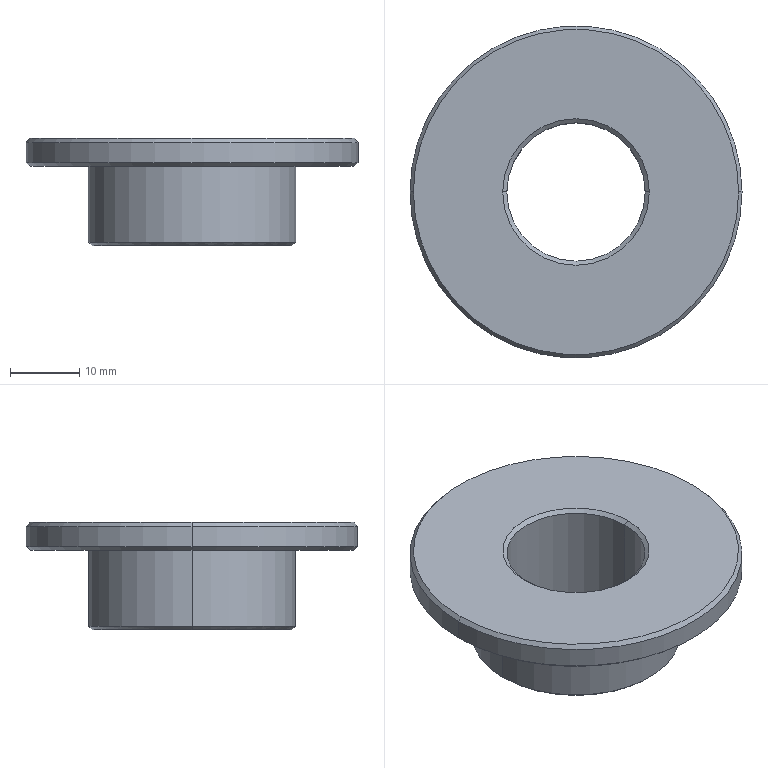Component | SolidWorks | CuttingMotorFixedShaftSleeve-1 | 1 solid | 19 faces | box 48 x 48 x 15.5 mm | volume 10420 mm3 | cone 10 | cylinder 6 | plane 3 | commonest cylinder face diameters 20 x2 30 x2 48 x2
build123d program:
from build123d import *
from OCP.BRepFilletAPI import BRepFilletAPI_MakeChamfer

# Parameters (mm, degrees)
CHAMFER1_SIZE  = 0.5
CHAMFER1_SIZE2 = 0.5959


with BuildPart() as part:
    # Sketch1 → Revolve1 (revolve)
    with BuildSketch(Plane.XY):
        Polygon((24, 0), (24, -4), (15, -4), (15, -15.5), (10, -15.5), (10, 0), align=None)
    revolve(axis=Axis((0, -1263.669, 0), (0, 1, 0)))

    # Chamfer1: one chamfer whose edges measure the first distance from different faces: ONE call of the kernel's chamfer builder (chamfer() names one face for all edges)
    chamfer1_edges_1 = [part.edges().sort_by_distance(p)[0] for p in [
        (-10, 0, 0),
    ]]
    chamfer1_side_1 = [part.faces().sort_by_distance(p)[0] for p in [
        (-10, -7.75, 0),
    ]]
    chamfer1_edges_2 = [part.edges().sort_by_distance(p)[0] for p in [
        (-10, -15.5, 0),
    ]]
    chamfer1_side_2 = [part.faces().sort_by_distance(p)[0] for p in [
        (-14.576, -15.5, 0),
    ]]
    chamfer1_edges_3 = [part.edges().sort_by_distance(p)[0] for p in [
        (-15, -15.5, 0),
    ]]
    chamfer1_side_3 = [part.faces().sort_by_distance(p)[0] for p in [
        (-15, -9.75, 0),
    ]]
    chamfer1_edges_4 = [part.edges().sort_by_distance(p)[0] for p in [
        (-24, -4, 0),
    ]]
    chamfer1_side_4 = [part.faces().sort_by_distance(p)[0] for p in [
        (-24, -2, 0),
    ]]
    chamfer1_edges_5 = [part.edges().sort_by_distance(p)[0] for p in [
        (-24, 0, 0),
    ]]
    chamfer1_side_5 = [part.faces().sort_by_distance(p)[0] for p in [
        (-10.679, 0, 0),
    ]]
    chamfer1 = BRepFilletAPI_MakeChamfer(part.part.solid().wrapped)
    for e in chamfer1_edges_1:
        chamfer1.Add(CHAMFER1_SIZE, CHAMFER1_SIZE2, e.wrapped, chamfer1_side_1[0].wrapped)  # the first distance lies on this face
    for e in chamfer1_edges_2:
        chamfer1.Add(CHAMFER1_SIZE, CHAMFER1_SIZE2, e.wrapped, chamfer1_side_2[0].wrapped)  # the first distance lies on this face
    for e in chamfer1_edges_3:
        chamfer1.Add(CHAMFER1_SIZE, CHAMFER1_SIZE2, e.wrapped, chamfer1_side_3[0].wrapped)  # the first distance lies on this face
    for e in chamfer1_edges_4:
        chamfer1.Add(CHAMFER1_SIZE, CHAMFER1_SIZE2, e.wrapped, chamfer1_side_4[0].wrapped)  # the first distance lies on this face
    for e in chamfer1_edges_5:
        chamfer1.Add(CHAMFER1_SIZE, CHAMFER1_SIZE2, e.wrapped, chamfer1_side_5[0].wrapped)  # the first distance lies on this face
    add(Compound.cast(chamfer1.Shape()), mode=Mode.REPLACE)


solid = part.part

# Placed as in the assembly
solid = solid.moved(Location((-22.772, -46.766, 806), (90, 0, 0)))
STEP:
#1=COLOUR_RGB('',0.7922,0.8196,0.9333);
#2=FILL_AREA_STYLE_COLOUR('',#1);
#3=FILL_AREA_STYLE('',(#2));
#4=SURFACE_STYLE_FILL_AREA(#3);
#5=SURFACE_SIDE_STYLE('',(#4));
#6=SURFACE_STYLE_USAGE(.BOTH.,#5);
#7=PRESENTATION_STYLE_ASSIGNMENT((#6));
#8=CARTESIAN_POINT('',(-1.822,-1.841,31.732));
#9=VERTEX_POINT('',#8);
#10=CARTESIAN_POINT('',(0.02866,-1.841,31.732));
#11=VERTEX_POINT('',#10);
#12=CARTESIAN_POINT('',(-0.8965,-1.841,31.732));
#13=DIRECTION('',(0.,-0.,1.));
#14=DIRECTION('',(-1.,-0.,0.));
#15=AXIS2_PLACEMENT_3D('',#12,#13,#14);
#16=CIRCLE('',#15,0.9252);
#17=EDGE_CURVE('',#9,#11,#16,.T.);
#18=ORIENTED_EDGE('',*,*,#17,.F.);
#19=CARTESIAN_POINT('',(-1.841,-1.841,31.709));
#20=VERTEX_POINT('',#19);
#21=CARTESIAN_POINT('',(-1.841,-1.841,31.709));
#22=DIRECTION('',(-0.6428,-0.,-0.766));
#23=VECTOR('',#22,39.37);
#24=LINE('',#21,#23);
#25=EDGE_CURVE('',#9,#20,#24,.T.);
#26=ORIENTED_EDGE('',*,*,#25,.T.);
#27=CARTESIAN_POINT('',(0.04834,-1.841,31.709));
#28=VERTEX_POINT('',#27);
#29=CARTESIAN_POINT('',(-0.8965,-1.841,31.709));
#30=DIRECTION('',(-0.,0.,-1.));
#31=DIRECTION('',(-1.,-0.,0.));
#32=AXIS2_PLACEMENT_3D('',#29,#30,#31);
#33=CIRCLE('',#32,0.9449);
#34=EDGE_CURVE('',#28,#20,#33,.T.);
#35=ORIENTED_EDGE('',*,*,#34,.F.);
#36=CARTESIAN_POINT('',(0.04834,-1.841,31.709));
#37=DIRECTION('',(0.6428,0.,-0.766));
#38=VECTOR('',#37,39.37);
#39=LINE('',#36,#38);
#40=EDGE_CURVE('',#11,#28,#39,.T.);
#41=ORIENTED_EDGE('',*,*,#40,.F.);
#42=EDGE_LOOP('',(#18,#26,#35,#41));
#43=FACE_OUTER_BOUND('',#42,.T.);
#44=CARTESIAN_POINT('',(-0.8965,-1.841,31.709));
#45=DIRECTION('',(-0.,0.,-1.));
#46=DIRECTION('',(1.,0.,0.));
#47=AXIS2_PLACEMENT_3D('',#44,#45,#46);
#48=CONICAL_SURFACE('',#47,0.9449,0.6981);
#49=ADVANCED_FACE('',(#43),#48,.T.);
#50=CARTESIAN_POINT('',(0.02488,-1.841,31.575));
#51=VERTEX_POINT('',#50);
#52=CARTESIAN_POINT('',(-1.818,-1.841,31.575));
#53=VERTEX_POINT('',#52);
#54=CARTESIAN_POINT('',(-0.8965,-1.841,31.575));
#55=DIRECTION('',(-0.,0.,-1.));
#56=DIRECTION('',(1.,0.,0.));
#57=AXIS2_PLACEMENT_3D('',#54,#55,#56);
#58=CIRCLE('',#57,0.9214);
#59=EDGE_CURVE('',#51,#53,#58,.T.);
#60=ORIENTED_EDGE('',*,*,#59,.F.);
#61=CARTESIAN_POINT('',(0.04834,-1.841,31.594));
#62=VERTEX_POINT('',#61);
#63=CARTESIAN_POINT('',(0.02488,-1.841,31.575));
#64=DIRECTION('',(0.766,0.,0.6428));
#65=VECTOR('',#64,39.37);
#66=LINE('',#63,#65);
#67=EDGE_CURVE('',#51,#62,#66,.T.);
#68=ORIENTED_EDGE('',*,*,#67,.T.);
#69=CARTESIAN_POINT('',(-1.841,-1.841,31.594));
#70=VERTEX_POINT('',#69);
#71=CARTESIAN_POINT('',(-0.8965,-1.841,31.594));
#72=DIRECTION('',(0.,-0.,1.));
#73=DIRECTION('',(1.,0.,0.));
#74=AXIS2_PLACEMENT_3D('',#71,#72,#73);
#75=CIRCLE('',#74,0.9449);
#76=EDGE_CURVE('',#70,#62,#75,.T.);
#77=ORIENTED_EDGE('',*,*,#76,.F.);
#78=CARTESIAN_POINT('',(-1.818,-1.841,31.575));
#79=DIRECTION('',(-0.766,-0.,0.6428));
#80=VECTOR('',#79,39.37);
#81=LINE('',#78,#80);
#82=EDGE_CURVE('',#53,#70,#81,.T.);
#83=ORIENTED_EDGE('',*,*,#82,.F.);
#84=EDGE_LOOP('',(#60,#68,#77,#83));
#85=FACE_OUTER_BOUND('',#84,.T.);
#86=CARTESIAN_POINT('',(-0.8965,-1.841,31.575));
#87=DIRECTION('',(0.,-0.,1.));
#88=DIRECTION('',(-1.,-0.,0.));
#89=AXIS2_PLACEMENT_3D('',#86,#87,#88);
#90=CONICAL_SURFACE('',#89,0.9214,0.8727);
#91=ADVANCED_FACE('',(#85),#90,.T.);
#92=CARTESIAN_POINT('',(-0.3294,-1.841,31.122));
#93=VERTEX_POINT('',#92);
#94=CARTESIAN_POINT('',(-1.464,-1.841,31.122));
#95=VERTEX_POINT('',#94);
#96=CARTESIAN_POINT('',(-0.8965,-1.841,31.122));
#97=DIRECTION('',(-0.,0.,-1.));
#98=DIRECTION('',(1.,0.,0.));
#99=AXIS2_PLACEMENT_3D('',#96,#97,#98);
#100=CIRCLE('',#99,0.5671);
#101=EDGE_CURVE('',#93,#95,#100,.T.);
#102=ORIENTED_EDGE('',*,*,#101,.F.);
#103=CARTESIAN_POINT('',(-0.306,-1.841,31.142));
#104=VERTEX_POINT('',#103);
#105=CARTESIAN_POINT('',(-0.3294,-1.841,31.122));
#106=DIRECTION('',(0.766,0.,0.6428));
#107=VECTOR('',#106,39.37);
#108=LINE('',#105,#107);
#109=EDGE_CURVE('',#93,#104,#108,.T.);
#110=ORIENTED_EDGE('',*,*,#109,.T.);
#111=CARTESIAN_POINT('',(-1.487,-1.841,31.142));
#112=VERTEX_POINT('',#111);
#113=CARTESIAN_POINT('',(-0.8965,-1.841,31.142));
#114=DIRECTION('',(0.,-0.,1.));
#115=DIRECTION('',(1.,0.,0.));
#116=AXIS2_PLACEMENT_3D('',#113,#114,#115);
#117=CIRCLE('',#116,0.5906);
#118=EDGE_CURVE('',#112,#104,#117,.T.);
#119=ORIENTED_EDGE('',*,*,#118,.F.);
#120=CARTESIAN_POINT('',(-1.464,-1.841,31.122));
#121=DIRECTION('',(-0.766,-0.,0.6428));
#122=VECTOR('',#121,39.37);
#123=LINE('',#120,#122);
#124=EDGE_CURVE('',#95,#112,#123,.T.);
#125=ORIENTED_EDGE('',*,*,#124,.F.);
#126=EDGE_LOOP('',(#102,#110,#119,#125));
#127=FACE_OUTER_BOUND('',#126,.T.);
#128=CARTESIAN_POINT('',(-0.8965,-1.841,31.122));
#129=DIRECTION('',(0.,-0.,1.));
#130=DIRECTION('',(-1.,-0.,0.));
#131=AXIS2_PLACEMENT_3D('',#128,#129,#130);
#132=CONICAL_SURFACE('',#131,0.5671,0.8727);
#133=ADVANCED_FACE('',(#127),#132,.T.);
#134=CARTESIAN_POINT('',(-1.29,-1.841,31.146));
#135=VERTEX_POINT('',#134);
#136=CARTESIAN_POINT('',(-0.5028,-1.841,31.146));
#137=VERTEX_POINT('',#136);
#138=CARTESIAN_POINT('',(-0.8965,-1.841,31.146));
#139=DIRECTION('',(-0.,0.,-1.));
#140=DIRECTION('',(1.,0.,0.));
#141=AXIS2_PLACEMENT_3D('',#138,#139,#140);
#142=CIRCLE('',#141,0.3937);
#143=EDGE_CURVE('',#135,#137,#142,.T.);
#144=ORIENTED_EDGE('',*,*,#143,.F.);
#145=CARTESIAN_POINT('',(-1.31,-1.841,31.122));
#146=VERTEX_POINT('',#145);
#147=CARTESIAN_POINT('',(-1.29,-1.841,31.146));
#148=DIRECTION('',(-0.6428,-0.,-0.766));
#149=VECTOR('',#148,39.37);
#150=LINE('',#147,#149);
#151=EDGE_CURVE('',#135,#146,#150,.T.);
#152=ORIENTED_EDGE('',*,*,#151,.T.);
#153=CARTESIAN_POINT('',(-0.4832,-1.841,31.122));
#154=VERTEX_POINT('',#153);
#155=CARTESIAN_POINT('',(-0.8965,-1.841,31.122));
#156=DIRECTION('',(0.,-0.,1.));
#157=DIRECTION('',(1.,0.,0.));
#158=AXIS2_PLACEMENT_3D('',#155,#156,#157);
#159=CIRCLE('',#158,0.4134);
#160=EDGE_CURVE('',#154,#146,#159,.T.);
#161=ORIENTED_EDGE('',*,*,#160,.F.);
#162=CARTESIAN_POINT('',(-0.5028,-1.841,31.146));
#163=DIRECTION('',(0.6428,0.,-0.766));
#164=VECTOR('',#163,39.37);
#165=LINE('',#162,#164);
#166=EDGE_CURVE('',#137,#154,#165,.T.);
#167=ORIENTED_EDGE('',*,*,#166,.F.);
#168=EDGE_LOOP('',(#144,#152,#161,#167));
#169=FACE_OUTER_BOUND('',#168,.T.);
#170=CARTESIAN_POINT('',(-0.8965,-1.841,31.146));
#171=DIRECTION('',(-0.,0.,-1.));
#172=DIRECTION('',(1.,0.,0.));
#173=AXIS2_PLACEMENT_3D('',#170,#171,#172);
#174=CONICAL_SURFACE('',#173,0.3937,0.6981);
#175=ADVANCED_FACE('',(#169),#174,.F.);
#176=CARTESIAN_POINT('',(-0.5028,-1.841,31.713));
#177=VERTEX_POINT('',#176);
#178=CARTESIAN_POINT('',(-1.29,-1.841,31.713));
#179=VERTEX_POINT('',#178);
#180=CARTESIAN_POINT('',(-0.8965,-1.841,31.713));
#181=DIRECTION('',(0.,-0.,1.));
#182=DIRECTION('',(-1.,-0.,0.));
#183=AXIS2_PLACEMENT_3D('',#180,#181,#182);
#184=CIRCLE('',#183,0.3937);
#185=EDGE_CURVE('',#177,#179,#184,.T.);
#186=ORIENTED_EDGE('',*,*,#185,.F.);
#187=CARTESIAN_POINT('',(-0.4794,-1.841,31.732));
#188=VERTEX_POINT('',#187);
#189=CARTESIAN_POINT('',(-0.4794,-1.841,31.732));
#190=DIRECTION('',(0.766,0.,0.6428));
#191=VECTOR('',#190,39.37);
#192=LINE('',#189,#191);
#193=EDGE_CURVE('',#177,#188,#192,.T.);
#194=ORIENTED_EDGE('',*,*,#193,.T.);
#195=CARTESIAN_POINT('',(-1.314,-1.841,31.732));
#196=VERTEX_POINT('',#195);
#197=CARTESIAN_POINT('',(-0.8965,-1.841,31.732));
#198=DIRECTION('',(-0.,0.,-1.));
#199=DIRECTION('',(-1.,-0.,0.));
#200=AXIS2_PLACEMENT_3D('',#197,#198,#199);
#201=CIRCLE('',#200,0.4172);
#202=EDGE_CURVE('',#196,#188,#201,.T.);
#203=ORIENTED_EDGE('',*,*,#202,.F.);
#204=CARTESIAN_POINT('',(-1.314,-1.841,31.732));
#205=DIRECTION('',(-0.766,-0.,0.6428));
#206=VECTOR('',#205,39.37);
#207=LINE('',#204,#206);
#208=EDGE_CURVE('',#179,#196,#207,.T.);
#209=ORIENTED_EDGE('',*,*,#208,.F.);
#210=EDGE_LOOP('',(#186,#194,#203,#209));
#211=FACE_OUTER_BOUND('',#210,.T.);
#212=CARTESIAN_POINT('',(-0.8965,-1.841,31.732));
#213=DIRECTION('',(0.,-0.,1.));
#214=DIRECTION('',(-1.,-0.,0.));
#215=AXIS2_PLACEMENT_3D('',#212,#213,#214);
#216=CONICAL_SURFACE('',#215,0.4172,0.8727);
#217=ADVANCED_FACE('',(#211),#216,.F.);
#218=ORIENTED_EDGE('',*,*,#185,.T.);
#219=CARTESIAN_POINT('',(-1.29,-1.841,-18.018));
#220=DIRECTION('',(-0.,0.,-1.));
#221=VECTOR('',#220,39.37);
#222=LINE('',#219,#221);
#223=EDGE_CURVE('',#179,#135,#222,.T.);
#224=ORIENTED_EDGE('',*,*,#223,.T.);
#225=ORIENTED_EDGE('',*,*,#143,.T.);
#226=CARTESIAN_POINT('',(-0.5028,-1.841,-18.018));
#227=DIRECTION('',(-0.,0.,-1.));
#228=VECTOR('',#227,39.37);
#229=LINE('',#226,#228);
#230=EDGE_CURVE('',#177,#137,#229,.T.);
#231=ORIENTED_EDGE('',*,*,#230,.F.);
#232=EDGE_LOOP('',(#218,#224,#225,#231));
#233=FACE_OUTER_BOUND('',#232,.T.);
#234=CARTESIAN_POINT('',(-0.8965,-1.841,-18.018));
#235=DIRECTION('',(-0.,0.,-1.));
#236=DIRECTION('',(1.,0.,0.));
#237=AXIS2_PLACEMENT_3D('',#234,#235,#236);
#238=CYLINDRICAL_SURFACE('',#237,0.3937);
#239=ADVANCED_FACE('',(#233),#238,.F.);
#240=CARTESIAN_POINT('',(-0.306,-1.841,31.575));
#241=VERTEX_POINT('',#240);
#242=CARTESIAN_POINT('',(-1.487,-1.841,31.575));
#243=VERTEX_POINT('',#242);
#244=CARTESIAN_POINT('',(-0.8965,-1.841,31.575));
#245=DIRECTION('',(-0.,0.,-1.));
#246=DIRECTION('',(1.,0.,0.));
#247=AXIS2_PLACEMENT_3D('',#244,#245,#246);
#248=CIRCLE('',#247,0.5906);
#249=EDGE_CURVE('',#241,#243,#248,.T.);
#250=ORIENTED_EDGE('',*,*,#249,.T.);
#251=CARTESIAN_POINT('',(-1.487,-1.841,-18.018));
#252=DIRECTION('',(-0.,0.,-1.));
#253=VECTOR('',#252,39.37);
#254=LINE('',#251,#253);
#255=EDGE_CURVE('',#243,#112,#254,.T.);
#256=ORIENTED_EDGE('',*,*,#255,.T.);
#257=ORIENTED_EDGE('',*,*,#118,.T.);
#258=CARTESIAN_POINT('',(-0.306,-1.841,-18.018));
#259=DIRECTION('',(-0.,0.,-1.));
#260=VECTOR('',#259,39.37);
#261=LINE('',#258,#260);
#262=EDGE_CURVE('',#241,#104,#261,.T.);
#263=ORIENTED_EDGE('',*,*,#262,.F.);
#264=EDGE_LOOP('',(#250,#256,#257,#263));
#265=FACE_OUTER_BOUND('',#264,.T.);
#266=CARTESIAN_POINT('',(-0.8965,-1.841,-18.018));
#267=DIRECTION('',(-0.,0.,-1.));
#268=DIRECTION('',(1.,0.,0.));
#269=AXIS2_PLACEMENT_3D('',#266,#267,#268);
#270=CYLINDRICAL_SURFACE('',#269,0.5906);
#271=ADVANCED_FACE('',(#265),#270,.T.);
#272=ORIENTED_EDGE('',*,*,#34,.T.);
#273=CARTESIAN_POINT('',(-1.841,-1.841,-18.018));
#274=DIRECTION('',(-0.,0.,-1.));
#275=VECTOR('',#274,39.37);
#276=LINE('',#273,#275);
#277=EDGE_CURVE('',#20,#70,#276,.T.);
#278=ORIENTED_EDGE('',*,*,#277,.T.);
#279=ORIENTED_EDGE('',*,*,#76,.T.);
#280=CARTESIAN_POINT('',(0.04834,-1.841,-18.018));
#281=DIRECTION('',(-0.,0.,-1.));
#282=VECTOR('',#281,39.37);
#283=LINE('',#280,#282);
#284=EDGE_CURVE('',#28,#62,#283,.T.);
#285=ORIENTED_EDGE('',*,*,#284,.F.);
#286=EDGE_LOOP('',(#272,#278,#279,#285));
#287=FACE_OUTER_BOUND('',#286,.T.);
#288=CARTESIAN_POINT('',(-0.8965,-1.841,-18.018));
#289=DIRECTION('',(-0.,0.,-1.));
#290=DIRECTION('',(1.,0.,0.));
#291=AXIS2_PLACEMENT_3D('',#288,#289,#290);
#292=CYLINDRICAL_SURFACE('',#291,0.9449);
#293=ADVANCED_FACE('',(#287),#292,.T.);
#294=ORIENTED_EDGE('',*,*,#202,.T.);
#295=CARTESIAN_POINT('',(-0.8965,-1.841,31.732));
#296=DIRECTION('',(-0.,0.,-1.));
#297=DIRECTION('',(-1.,-0.,0.));
#298=AXIS2_PLACEMENT_3D('',#295,#296,#297);
#299=CIRCLE('',#298,0.4172);
#300=EDGE_CURVE('',#188,#196,#299,.T.);
#301=ORIENTED_EDGE('',*,*,#300,.T.);
#302=EDGE_LOOP('',(#294,#301));
#303=FACE_BOUND('',#302,.T.);
#304=CARTESIAN_POINT('',(-0.8965,-1.841,31.732));
#305=DIRECTION('',(0.,-0.,1.));
#306=DIRECTION('',(-1.,-0.,0.));
#307=AXIS2_PLACEMENT_3D('',#304,#305,#306);
#308=CIRCLE('',#307,0.9252);
#309=EDGE_CURVE('',#11,#9,#308,.T.);
#310=ORIENTED_EDGE('',*,*,#309,.T.);
#311=ORIENTED_EDGE('',*,*,#17,.T.);
#312=EDGE_LOOP('',(#310,#311));
#313=FACE_OUTER_BOUND('',#312,.T.);
#314=CARTESIAN_POINT('',(-0.5028,-1.841,31.732));
#315=DIRECTION('',(0.,-0.,1.));
#316=DIRECTION('',(-1.,-0.,0.));
#317=AXIS2_PLACEMENT_3D('',#314,#315,#316);
#318=PLANE('',#317);
#319=ADVANCED_FACE('',(#303,#313),#318,.T.);
#320=ORIENTED_EDGE('',*,*,#277,.F.);
#321=CARTESIAN_POINT('',(-0.8965,-1.841,31.709));
#322=DIRECTION('',(-0.,0.,-1.));
#323=DIRECTION('',(-1.,-0.,0.));
#324=AXIS2_PLACEMENT_3D('',#321,#322,#323);
#325=CIRCLE('',#324,0.9449);
#326=EDGE_CURVE('',#20,#28,#325,.T.);
#327=ORIENTED_EDGE('',*,*,#326,.T.);
#328=ORIENTED_EDGE('',*,*,#284,.T.);
#329=CARTESIAN_POINT('',(-0.8965,-1.841,31.594));
#330=DIRECTION('',(0.,-0.,1.));
#331=DIRECTION('',(1.,0.,0.));
#332=AXIS2_PLACEMENT_3D('',#329,#330,#331);
#333=CIRCLE('',#332,0.9449);
#334=EDGE_CURVE('',#62,#70,#333,.T.);
#335=ORIENTED_EDGE('',*,*,#334,.T.);
#336=EDGE_LOOP('',(#320,#327,#328,#335));
#337=FACE_OUTER_BOUND('',#336,.T.);
#338=CARTESIAN_POINT('',(-0.8965,-1.841,-18.018));
#339=DIRECTION('',(-0.,0.,-1.));
#340=DIRECTION('',(1.,0.,0.));
#341=AXIS2_PLACEMENT_3D('',#338,#339,#340);
#342=CYLINDRICAL_SURFACE('',#341,0.9449);
#343=ADVANCED_FACE('',(#337),#342,.T.);
#344=CARTESIAN_POINT('',(-0.8965,-1.841,31.575));
#345=DIRECTION('',(-0.,0.,-1.));
#346=DIRECTION('',(1.,0.,0.));
#347=AXIS2_PLACEMENT_3D('',#344,#345,#346);
#348=CIRCLE('',#347,0.9214);
#349=EDGE_CURVE('',#53,#51,#348,.T.);
#350=ORIENTED_EDGE('',*,*,#349,.T.);
#351=ORIENTED_EDGE('',*,*,#59,.T.);
#352=EDGE_LOOP('',(#350,#351));
#353=FACE_OUTER_BOUND('',#352,.T.);
#354=ORIENTED_EDGE('',*,*,#249,.F.);
#355=CARTESIAN_POINT('',(-0.8965,-1.841,31.575));
#356=DIRECTION('',(-0.,0.,-1.));
#357=DIRECTION('',(1.,0.,0.));
#358=AXIS2_PLACEMENT_3D('',#355,#356,#357);
#359=CIRCLE('',#358,0.5906);
#360=EDGE_CURVE('',#243,#241,#359,.T.);
#361=ORIENTED_EDGE('',*,*,#360,.F.);
#362=EDGE_LOOP('',(#354,#361));
#363=FACE_BOUND('',#362,.T.);
#364=CARTESIAN_POINT('',(0.04834,-1.841,31.575));
#365=DIRECTION('',(-0.,0.,-1.));
#366=DIRECTION('',(1.,0.,-0.));
#367=AXIS2_PLACEMENT_3D('',#364,#365,#366);
#368=PLANE('',#367);
#369=ADVANCED_FACE('',(#353,#363),#368,.T.);
#370=ORIENTED_EDGE('',*,*,#255,.F.);
#371=ORIENTED_EDGE('',*,*,#360,.T.);
#372=ORIENTED_EDGE('',*,*,#262,.T.);
#373=CARTESIAN_POINT('',(-0.8965,-1.841,31.142));
#374=DIRECTION('',(0.,-0.,1.));
#375=DIRECTION('',(1.,0.,0.));
#376=AXIS2_PLACEMENT_3D('',#373,#374,#375);
#377=CIRCLE('',#376,0.5906);
#378=EDGE_CURVE('',#104,#112,#377,.T.);
#379=ORIENTED_EDGE('',*,*,#378,.T.);
#380=EDGE_LOOP('',(#370,#371,#372,#379));
#381=FACE_OUTER_BOUND('',#380,.T.);
#382=CARTESIAN_POINT('',(-0.8965,-1.841,-18.018));
#383=DIRECTION('',(-0.,0.,-1.));
#384=DIRECTION('',(1.,0.,0.));
#385=AXIS2_PLACEMENT_3D('',#382,#383,#384);
#386=CYLINDRICAL_SURFACE('',#385,0.5906);
#387=ADVANCED_FACE('',(#381),#386,.T.);
#388=ORIENTED_EDGE('',*,*,#160,.T.);
#389=CARTESIAN_POINT('',(-0.8965,-1.841,31.122));
#390=DIRECTION('',(0.,-0.,1.));
#391=DIRECTION('',(1.,0.,0.));
#392=AXIS2_PLACEMENT_3D('',#389,#390,#391);
#393=CIRCLE('',#392,0.4134);
#394=EDGE_CURVE('',#146,#154,#393,.T.);
#395=ORIENTED_EDGE('',*,*,#394,.T.);
#396=EDGE_LOOP('',(#388,#395));
#397=FACE_BOUND('',#396,.T.);
#398=CARTESIAN_POINT('',(-0.8965,-1.841,31.122));
#399=DIRECTION('',(-0.,0.,-1.));
#400=DIRECTION('',(1.,0.,0.));
#401=AXIS2_PLACEMENT_3D('',#398,#399,#400);
#402=CIRCLE('',#401,0.5671);
#403=EDGE_CURVE('',#95,#93,#402,.T.);
#404=ORIENTED_EDGE('',*,*,#403,.T.);
#405=ORIENTED_EDGE('',*,*,#101,.T.);
#406=EDGE_LOOP('',(#404,#405));
#407=FACE_OUTER_BOUND('',#406,.T.);
#408=CARTESIAN_POINT('',(-0.306,-1.841,31.122));
#409=DIRECTION('',(-0.,0.,-1.));
#410=DIRECTION('',(1.,0.,-0.));
#411=AXIS2_PLACEMENT_3D('',#408,#409,#410);
#412=PLANE('',#411);
#413=ADVANCED_FACE('',(#397,#407),#412,.T.);
#414=ORIENTED_EDGE('',*,*,#223,.F.);
#415=CARTESIAN_POINT('',(-0.8965,-1.841,31.713));
#416=DIRECTION('',(0.,-0.,1.));
#417=DIRECTION('',(-1.,-0.,0.));
#418=AXIS2_PLACEMENT_3D('',#415,#416,#417);
#419=CIRCLE('',#418,0.3937);
#420=EDGE_CURVE('',#179,#177,#419,.T.);
#421=ORIENTED_EDGE('',*,*,#420,.T.);
#422=ORIENTED_EDGE('',*,*,#230,.T.);
#423=CARTESIAN_POINT('',(-0.8965,-1.841,31.146));
#424=DIRECTION('',(-0.,0.,-1.));
#425=DIRECTION('',(1.,0.,0.));
#426=AXIS2_PLACEMENT_3D('',#423,#424,#425);
#427=CIRCLE('',#426,0.3937);
#428=EDGE_CURVE('',#137,#135,#427,.T.);
#429=ORIENTED_EDGE('',*,*,#428,.T.);
#430=EDGE_LOOP('',(#414,#421,#422,#429));
#431=FACE_OUTER_BOUND('',#430,.T.);
#432=CARTESIAN_POINT('',(-0.8965,-1.841,-18.018));
#433=DIRECTION('',(-0.,0.,-1.));
#434=DIRECTION('',(1.,0.,0.));
#435=AXIS2_PLACEMENT_3D('',#432,#433,#434);
#436=CYLINDRICAL_SURFACE('',#435,0.3937);
#437=ADVANCED_FACE('',(#431),#436,.F.);
#438=ORIENTED_EDGE('',*,*,#193,.F.);
#439=ORIENTED_EDGE('',*,*,#420,.F.);
#440=ORIENTED_EDGE('',*,*,#208,.T.);
#441=ORIENTED_EDGE('',*,*,#300,.F.);
#442=EDGE_LOOP('',(#438,#439,#440,#441));
#443=FACE_OUTER_BOUND('',#442,.T.);
#444=CARTESIAN_POINT('',(-0.8965,-1.841,31.732));
#445=DIRECTION('',(0.,-0.,1.));
#446=DIRECTION('',(-1.,-0.,0.));
#447=AXIS2_PLACEMENT_3D('',#444,#445,#446);
#448=CONICAL_SURFACE('',#447,0.4172,0.8727);
#449=ADVANCED_FACE('',(#443),#448,.F.);
#450=ORIENTED_EDGE('',*,*,#151,.F.);
#451=ORIENTED_EDGE('',*,*,#428,.F.);
#452=ORIENTED_EDGE('',*,*,#166,.T.);
#453=ORIENTED_EDGE('',*,*,#394,.F.);
#454=EDGE_LOOP('',(#450,#451,#452,#453));
#455=FACE_OUTER_BOUND('',#454,.T.);
#456=CARTESIAN_POINT('',(-0.8965,-1.841,31.146));
#457=DIRECTION('',(-0.,0.,-1.));
#458=DIRECTION('',(1.,0.,0.));
#459=AXIS2_PLACEMENT_3D('',#456,#457,#458);
#460=CONICAL_SURFACE('',#459,0.3937,0.6981);
#461=ADVANCED_FACE('',(#455),#460,.F.);
#462=ORIENTED_EDGE('',*,*,#109,.F.);
#463=ORIENTED_EDGE('',*,*,#403,.F.);
#464=ORIENTED_EDGE('',*,*,#124,.T.);
#465=ORIENTED_EDGE('',*,*,#378,.F.);
#466=EDGE_LOOP('',(#462,#463,#464,#465));
#467=FACE_OUTER_BOUND('',#466,.T.);
#468=CARTESIAN_POINT('',(-0.8965,-1.841,31.122));
#469=DIRECTION('',(0.,-0.,1.));
#470=DIRECTION('',(-1.,-0.,0.));
#471=AXIS2_PLACEMENT_3D('',#468,#469,#470);
#472=CONICAL_SURFACE('',#471,0.5671,0.8727);
#473=ADVANCED_FACE('',(#467),#472,.T.);
#474=ORIENTED_EDGE('',*,*,#67,.F.);
#475=ORIENTED_EDGE('',*,*,#349,.F.);
#476=ORIENTED_EDGE('',*,*,#82,.T.);
#477=ORIENTED_EDGE('',*,*,#334,.F.);
#478=EDGE_LOOP('',(#474,#475,#476,#477));
#479=FACE_OUTER_BOUND('',#478,.T.);
#480=CARTESIAN_POINT('',(-0.8965,-1.841,31.575));
#481=DIRECTION('',(0.,-0.,1.));
#482=DIRECTION('',(-1.,-0.,0.));
#483=AXIS2_PLACEMENT_3D('',#480,#481,#482);
#484=CONICAL_SURFACE('',#483,0.9214,0.8727);
#485=ADVANCED_FACE('',(#479),#484,.T.);
#486=ORIENTED_EDGE('',*,*,#25,.F.);
#487=ORIENTED_EDGE('',*,*,#309,.F.);
#488=ORIENTED_EDGE('',*,*,#40,.T.);
#489=ORIENTED_EDGE('',*,*,#326,.F.);
#490=EDGE_LOOP('',(#486,#487,#488,#489));
#491=FACE_OUTER_BOUND('',#490,.T.);
#492=CARTESIAN_POINT('',(-0.8965,-1.841,31.709));
#493=DIRECTION('',(-0.,0.,-1.));
#494=DIRECTION('',(1.,0.,0.));
#495=AXIS2_PLACEMENT_3D('',#492,#493,#494);
#496=CONICAL_SURFACE('',#495,0.9449,0.6981);
#497=ADVANCED_FACE('',(#491),#496,.T.);
#498=CLOSED_SHELL('',(#49,#91,#133,#175,#217,#239,#271,#293,#319,#343,#369,#387,#413,#437,#449,#461,#473,#485,#497));
#499=MANIFOLD_SOLID_BREP('',#498);
#500=STYLED_ITEM('',(#7),#499);
#501=PRESENTATION_LAYER_ASSIGNMENT('','',(#500));
#502=CARTESIAN_POINT('',(0.,0.,0.));
#503=DIRECTION('',(0.,0.,1.));
#504=DIRECTION('',(1.,0.,0.));
#505=AXIS2_PLACEMENT_3D('',#502,#503,#504);
#506=(LENGTH_UNIT()NAMED_UNIT(*)SI_UNIT($,.METRE.));
#507=LENGTH_MEASURE_WITH_UNIT(LENGTH_MEASURE(0.0254),#506);
#508=DIMENSIONAL_EXPONENTS(1.,0.,0.,0.,0.,0.,0.);
#509=(CONVERSION_BASED_UNIT('',#507)LENGTH_UNIT()NAMED_UNIT(#508));
#510=UNCERTAINTY_MEASURE_WITH_UNIT(LENGTH_MEASURE(0.00001),#509,'','');
#511=(NAMED_UNIT(*)PLANE_ANGLE_UNIT()SI_UNIT($,.RADIAN.));
#512=(NAMED_UNIT(*)SI_UNIT($,.STERADIAN.)SOLID_ANGLE_UNIT());
#513=(GEOMETRIC_REPRESENTATION_CONTEXT(3)GLOBAL_UNCERTAINTY_ASSIGNED_CONTEXT((#510))GLOBAL_UNIT_ASSIGNED_CONTEXT((#509,#511,#512))REPRESENTATION_CONTEXT('',''));
#514=ADVANCED_BREP_SHAPE_REPRESENTATION('',(#499,#505),#513);
#515=(LENGTH_UNIT()NAMED_UNIT(*)SI_UNIT($,.METRE.));
#516=LENGTH_MEASURE_WITH_UNIT(LENGTH_MEASURE(0.0254),#515);
#517=DIMENSIONAL_EXPONENTS(1.,0.,0.,0.,0.,0.,0.);
#518=(CONVERSION_BASED_UNIT('',#516)LENGTH_UNIT()NAMED_UNIT(#517));
#519=UNCERTAINTY_MEASURE_WITH_UNIT(LENGTH_MEASURE(0.00001),#518,'','');
#520=(NAMED_UNIT(*)PLANE_ANGLE_UNIT()SI_UNIT($,.RADIAN.));
#521=(NAMED_UNIT(*)SI_UNIT($,.STERADIAN.)SOLID_ANGLE_UNIT());
#522=(GEOMETRIC_REPRESENTATION_CONTEXT(3)GLOBAL_UNCERTAINTY_ASSIGNED_CONTEXT((#519))GLOBAL_UNIT_ASSIGNED_CONTEXT((#518,#520,#521))REPRESENTATION_CONTEXT('',''));
#523=MECHANICAL_DESIGN_GEOMETRIC_PRESENTATION_REPRESENTATION('',(#500),#522);